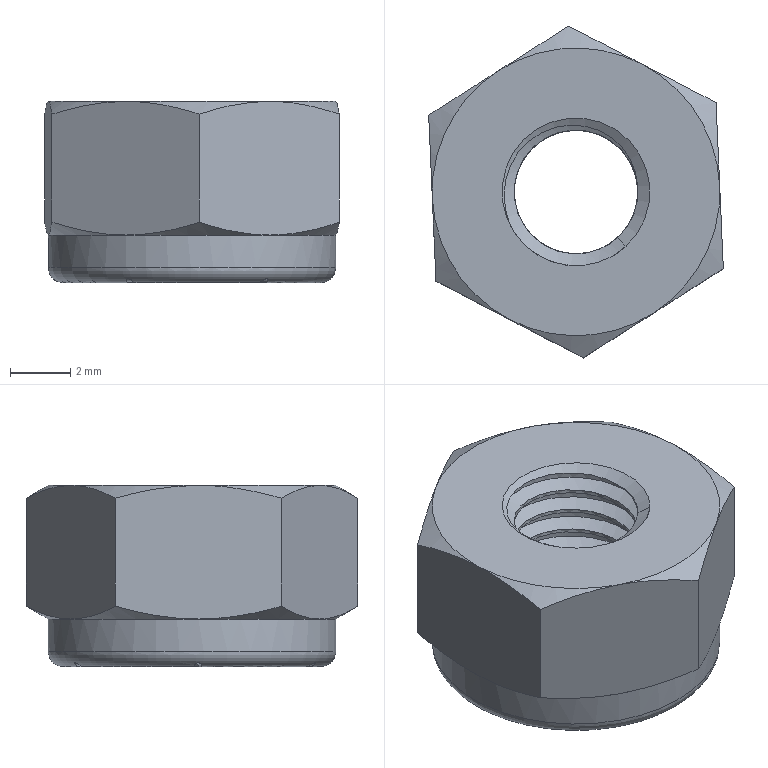Component | NX | MOUNTINGNUT_2 | 1 solid | 49 faces | volume 358 mm3 | plane 19 | cone 15 | cylinder 10 | spline 4 | torus 1 | commonest cylinder face diameters 0.25 x6 4.894 x2 9.525 x1 4.1 x1